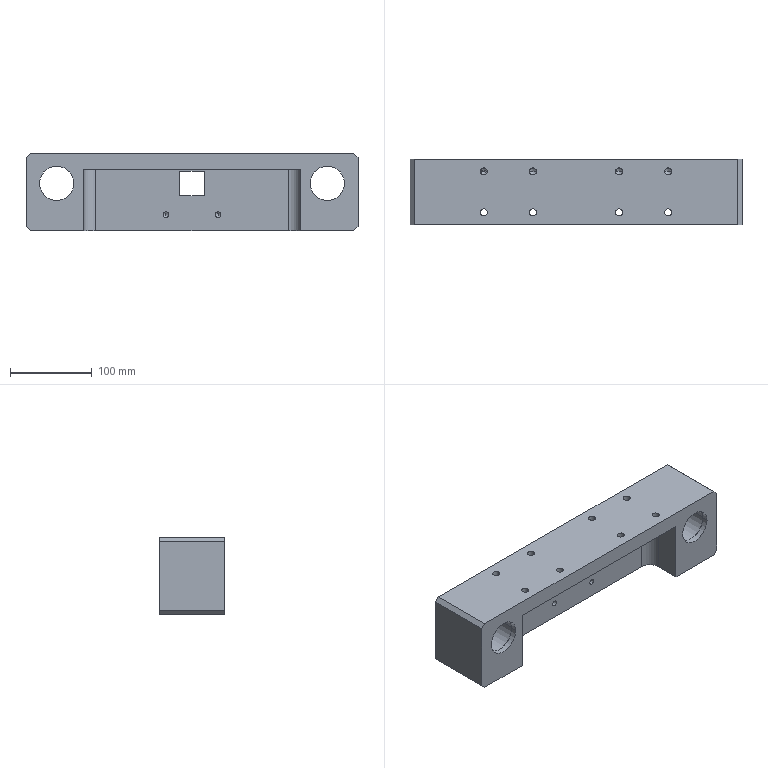Component | SolidWorks | GuidePostMountingPlate-1 | 1 solid | 100 faces | box 405 x 80 x 95 mm | volume 1862281 mm3 | cylinder 50 | cone 28 | plane 22 | commonest cylinder face diameters 6.8 x20 8.5 x16 42 x4 44 x4 60 x4 30 x2 | material 1023 Carbon Steel Plate (SS)
build123d program:
from build123d import *

# Parameters (mm, degrees)
SKETCH1_W                   = 405
SKETCH1_H                   = 80
BOSS_EXTRUDE1_DEPTH         = 47.5
SKETCH2_W                   = 265
SKETCH2_H                   = 45
CUT_EXTRUDE1_DEPTH          = 75
FILLET1_R                   = 15
SKETCH3_R                   = 22
CUT_EXTRUDE2_DEPTH          = 73
SKETCH4_W                   = 30
SKETCH4_H                   = 30
CUT_EXTRUDE3_DEPTH          = 76
SKETCH5_R                   = 30
CUT_EXTRUDE4_DEPTH          = 13
SKETCH7_R                   = 21
CUT_EXTRUDE5_DEPTH          = 221.435
CIRPATTERN1_COUNT           = 4
M8_TAPPED_HOLE2_D           = 6.8
M8_TAPPED_HOLE2_DEPTH       = 19.75
M8_TAPPED_HOLE2_TIP         = 2.043
M10_TAPPED_HOLE1_AT_2_COUNT = 2
M10_TAPPED_HOLE1_AT_2_PITCH = 60
M10_TAPPED_HOLE1_AT_3_COUNT = 2
M10_TAPPED_HOLE1_AT_3_PITCH = 105
M10_TAPPED_HOLE1_AT_4_COUNT = 2
M10_TAPPED_HOLE1_AT_4_PITCH = 165
CHAMFER1_SIZE               = 5


with BuildPart() as part:
    # Sketch1 → Boss-Extrude1 (new, symmetric)
    with BuildSketch(Plane.XY):
        Rectangle(SKETCH1_W, SKETCH1_H)
    extrude(amount=BOSS_EXTRUDE1_DEPTH, both=True)

    # Sketch2 → Cut-Extrude1 (cut)
    with BuildSketch(Plane.XY.offset(47.5)):
        with Locations((0, -17.5)):
            Rectangle(SKETCH2_W, SKETCH2_H)
    extrude(amount=-CUT_EXTRUDE1_DEPTH, mode=Mode.SUBTRACT)

    # Fillet1
    fillet1_edges = [part.edges().sort_by_distance(p)[0] for p in [
        (-132.5, 5, 10),
        (132.5, 5, 10),
    ]]
    fillet(fillet1_edges, radius=FILLET1_R)

    # Sketch3 → Cut-Extrude2 (cut)
    with BuildSketch(Plane(origin=(0, 40, 0), x_dir=(1, 0, 0), z_dir=(0, 1, 0))):
        with Locations(Location((-165, 10.5, 0), (0, 0, 180))):
            Circle(SKETCH3_R)
        with Locations(Location((165, 10.5, 0), (0, 0, 180))):
            Circle(SKETCH3_R)
    extrude(amount=-CUT_EXTRUDE2_DEPTH, mode=Mode.SUBTRACT)

    # Sketch4 → Cut-Extrude3 (cut)
    with BuildSketch(Plane(origin=(0, 40, 0), x_dir=(1, 0, 0), z_dir=(0, 1, 0))):
        with Locations((0, 10.5)):
            Rectangle(SKETCH4_W, SKETCH4_H)
    extrude(amount=-CUT_EXTRUDE3_DEPTH, mode=Mode.SUBTRACT)

    # Sketch5 → Cut-Extrude4 (cut)
    with BuildSketch(Plane(origin=(0, 40, 0), x_dir=(1, 0, 0), z_dir=(0, 1, 0))):
        with Locations(Location((-165, 10.5, 0), (0, 0, 180))):
            Circle(SKETCH5_R)
    cut_extrude4 = extrude(amount=-CUT_EXTRUDE4_DEPTH, mode=Mode.SUBTRACT)

    # Sketch7 → Cut-Extrude5 (cut, through all)
    with BuildSketch(Plane(origin=(0, -33, 0), x_dir=(1, 0, 0), z_dir=(0, 1, 0))):
        with Locations(Location((-165, 10.5, 0), (0, 0, 180))):
            Circle(SKETCH7_R)
    cut_extrude5 = extrude(amount=-CUT_EXTRUDE5_DEPTH, mode=Mode.SUBTRACT)

    # Mirror1: Cut-Extrude4, Cut-Extrude5 across plane
    add(cut_extrude4.mirror(Plane(origin=(0, 0, 0), x_dir=(0, 0, 1), z_dir=(1, 0, 0))), mode=Mode.SUBTRACT)
    add(cut_extrude5.mirror(Plane(origin=(0, 0, 0), x_dir=(0, 0, 1), z_dir=(1, 0, 0))), mode=Mode.SUBTRACT)

    # Sketch10 → M8 Tapped Hole1 (revolve, cut)
    with BuildSketch(Plane(origin=(-137.423, 40, -38.077), x_dir=(0, 0, 1), z_dir=(1, 0, 0))):
        Polygon((0, 0), (0, 21.793), (3.4, 19.75), (3.4, 0), align=None)
    m8_tapped_hole1 = revolve(axis=Axis((-137.423, 46.35, -38.077), (0, -1, 0)), mode=Mode.SUBTRACT)

    # CirPattern1: M8 Tapped Hole1 ×4 about axis
    cirpattern1_axis = Axis((-165, 0, -10.5), (0, 1, 0))
    for i in range(1, CIRPATTERN1_COUNT):
        add(m8_tapped_hole1.rotate(cirpattern1_axis, i * 360 / CIRPATTERN1_COUNT), mode=Mode.SUBTRACT)

    # Mirror2: M8 Tapped Hole1 across plane
    add(m8_tapped_hole1.mirror(Plane(origin=(0, 0, 0), x_dir=(0, 0, 1), z_dir=(1, 0, 0))), mode=Mode.SUBTRACT)

    # Mirror2 copy 1 sketch → Mirror2 copy 1 (revolve, cut)
    with BuildSketch(Plane(origin=(192.577, 40, -38.077), x_dir=(-1, 0, 0), z_dir=(0, 0, -1))):
        Polygon((0, 0), (0, -21.793), (3.4, -19.75), (3.4, 0), align=None)
    revolve(axis=Axis((192.577, 46.35, -38.077), (0, 1, 0)), mode=Mode.SUBTRACT)

    # Mirror2 copy 2 sketch → Mirror2 copy 2 (revolve, cut)
    with BuildSketch(Plane(origin=(192.577, 40, 17.077), x_dir=(0, 0, -1), z_dir=(1, 0, 0))):
        Polygon((0, 0), (0, -21.793), (3.4, -19.75), (3.4, 0), align=None)
    revolve(axis=Axis((192.577, 46.35, 17.077), (0, 1, 0)), mode=Mode.SUBTRACT)

    # Mirror2 copy 3 sketch → Mirror2 copy 3 (revolve, cut)
    with BuildSketch(Plane(origin=(137.423, 40, 17.077), x_dir=(1, 0, 0), z_dir=(0, 0, 1))):
        Polygon((0, 0), (0, -21.793), (3.4, -19.75), (3.4, 0), align=None)
    revolve(axis=Axis((137.423, 46.35, 17.077), (0, 1, 0)), mode=Mode.SUBTRACT)

    # M8 Tapped Hole2
    with Locations(Plane(origin=(0, 5, 0), x_dir=(-1, 0, 0), z_dir=(0, -1, 0))):
        with Locations((32, -27.5), (-32, -27.5)):
            Hole(M8_TAPPED_HOLE2_D / 2, depth=M8_TAPPED_HOLE2_DEPTH)
            with Locations((0, 0, -(M8_TAPPED_HOLE2_DEPTH + M8_TAPPED_HOLE2_TIP / 2))):  # 118° drill point
                Cone(0, M8_TAPPED_HOLE2_D / 2, M8_TAPPED_HOLE2_TIP, mode=Mode.SUBTRACT)

    # Sketch14 → M10 Tapped Hole1 (revolve, cut)
    with BuildSketch(Plane(origin=(-52.5, 25, -47.5), x_dir=(0, 1, 0), z_dir=(1, 0, 0))):
        Polygon((0, 0), (0, 27.054), (4.25, 24.5), (4.25, 0), align=None)
    m10_tapped_hole1 = revolve(axis=Axis((-52.5, 25, -53.85), (0, 0, 1)), mode=Mode.SUBTRACT)

    # M10 Tapped Hole1 at 2: M10 Tapped Hole1 ×2
    with Locations(*[(-i * M10_TAPPED_HOLE1_AT_2_PITCH, 0, 0) for i in range(1, M10_TAPPED_HOLE1_AT_2_COUNT)]):
        add(m10_tapped_hole1, mode=Mode.SUBTRACT)

    # M10 Tapped Hole1 at 3: M10 Tapped Hole1 ×2
    with Locations(*[(i * M10_TAPPED_HOLE1_AT_3_PITCH, 0, 0) for i in range(1, M10_TAPPED_HOLE1_AT_3_COUNT)]):
        add(m10_tapped_hole1, mode=Mode.SUBTRACT)

    # M10 Tapped Hole1 at 4: M10 Tapped Hole1 ×2
    with Locations(*[(i * M10_TAPPED_HOLE1_AT_4_PITCH, 0, 0) for i in range(1, M10_TAPPED_HOLE1_AT_4_COUNT)]):
        add(m10_tapped_hole1, mode=Mode.SUBTRACT)

    # Chamfer1
    chamfer1_edges = [part.edges().sort_by_distance(p)[0] for p in [
        (202.5, 0, 47.5),
        (-202.5, 0, 47.5),
        (202.5, 0, -47.5),
        (-202.5, 0, -47.5),
    ]]
    chamfer(chamfer1_edges, length=CHAMFER1_SIZE)

    # Mirror3: M10 Tapped Hole1 across plane
    add(m10_tapped_hole1.mirror(Plane.ZX), mode=Mode.SUBTRACT)

    # Mirror3 copy 1 sketch → Mirror3 copy 1 (revolve, cut)
    with BuildSketch(Plane(origin=(-112.5, -25, -47.5), x_dir=(0, -1, 0), z_dir=(1, 0, 0))):
        Polygon((0, 0), (0, -27.054), (4.25, -24.5), (4.25, 0), align=None)
    revolve(axis=Axis((-112.5, -25, -53.85), (0, 0, -1)), mode=Mode.SUBTRACT)

    # Mirror3 copy 2 sketch → Mirror3 copy 2 (revolve, cut)
    with BuildSketch(Plane(origin=(52.5, -25, -47.5), x_dir=(0, -1, 0), z_dir=(1, 0, 0))):
        Polygon((0, 0), (0, -27.054), (4.25, -24.5), (4.25, 0), align=None)
    revolve(axis=Axis((52.5, -25, -53.85), (0, 0, -1)), mode=Mode.SUBTRACT)

    # Mirror3 copy 3 sketch → Mirror3 copy 3 (revolve, cut)
    with BuildSketch(Plane(origin=(112.5, -25, -47.5), x_dir=(0, -1, 0), z_dir=(1, 0, 0))):
        Polygon((0, 0), (0, -27.054), (4.25, -24.5), (4.25, 0), align=None)
    revolve(axis=Axis((112.5, -25, -53.85), (0, 0, -1)), mode=Mode.SUBTRACT)


solid = part.part

# Placed as in the assembly
solid = solid.moved(Location((-29.507, -33.411, 447.5), (-180, 0, 180)))